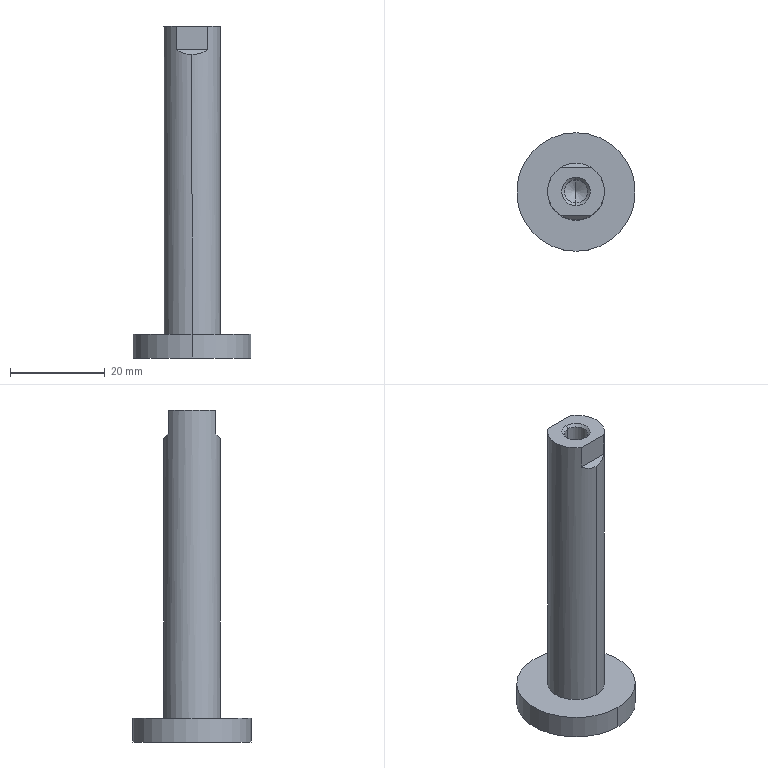Component | SolidWorks | CDQ2B25-50DZ-M9N(0_0_0)-1_CDQ2B25-50M9N(0_0)_CYROD-1 | 1 solid | 17 faces | box 25 x 25 x 70 mm | volume 9518 mm3 | plane 7 | cylinder 6 | cone 4 | commonest cylinder face diameters 25 x2 12 x2 4.917 x2
build123d program:
from build123d import *

# Parameters (mm, degrees)
EXTRUDE1_DEPTH      = 12
EXTRUDE1_DEPTH_BACK = 12


with BuildPart() as part:
    # Sketch1 → Revolve1 (revolve)
    with BuildSketch(Plane.XY, mode=Mode.PRIVATE) as revolve1_sk:
        Polygon((8.419, 0), (7, 2.458), (-4.458, 2.458), (-5, 3), (-5, 6), (60, 6), (60, 12.5), (65, 12.5), (65, 0), align=None)
    revolve(revolve1_sk.sketch.rotate(Axis((65, 0, 0), (-1, 0, 0)), 270), axis=Axis((65, 0, 0), (-1, 0, 0)))

    # Sketch2 → Extrude1 (cut, two sides: drawn at the far end of the back side and taken through both)
    with BuildSketch(Plane(origin=(0, 0, 0), x_dir=(1, 0, 0), z_dir=(0, 1, 0)).offset(-EXTRUDE1_DEPTH_BACK)):
        Polygon((-10, 10), (-10, -10), (5, -10), (0, -5), (-5, -5), (-5, 5), (0, 5), (5, 10), align=None)
    extrude(amount=EXTRUDE1_DEPTH + EXTRUDE1_DEPTH_BACK, mode=Mode.SUBTRACT)


solid = part.part

# Placed as in the assembly
solid = solid.moved(Location((0, -65.5, 248.966), (90, 0, -90)))
STEP:
#1=COLOUR_RGB('',0.7922,0.8196,0.9333);
#2=FILL_AREA_STYLE_COLOUR('',#1);
#3=FILL_AREA_STYLE('',(#2));
#4=SURFACE_STYLE_FILL_AREA(#3);
#5=SURFACE_SIDE_STYLE('',(#4));
#6=SURFACE_STYLE_USAGE(.BOTH.,#5);
#7=PRESENTATION_STYLE_ASSIGNMENT((#6));
#8=CARTESIAN_POINT('',(-0.,-3.071,7.243));
#9=VERTEX_POINT('',#8);
#10=CARTESIAN_POINT('',(-0.,-2.087,7.243));
#11=VERTEX_POINT('',#10);
#12=CARTESIAN_POINT('',(-0.,-2.579,7.243));
#13=DIRECTION('',(-0.,0.,1.));
#14=DIRECTION('',(0.,-1.,0.));
#15=AXIS2_PLACEMENT_3D('',#12,#13,#14);
#16=CIRCLE('',#15,0.4921);
#17=EDGE_CURVE('',#9,#11,#16,.T.);
#18=ORIENTED_EDGE('',*,*,#17,.T.);
#19=CARTESIAN_POINT('',(-0.,-2.087,7.44));
#20=VERTEX_POINT('',#19);
#21=CARTESIAN_POINT('',(-0.,-2.087,7.243));
#22=DIRECTION('',(-0.,0.,1.));
#23=VECTOR('',#22,39.37);
#24=LINE('',#21,#23);
#25=EDGE_CURVE('',#11,#20,#24,.T.);
#26=ORIENTED_EDGE('',*,*,#25,.T.);
#27=CARTESIAN_POINT('',(-0.,-3.071,7.44));
#28=VERTEX_POINT('',#27);
#29=CARTESIAN_POINT('',(-0.,-2.579,7.44));
#30=DIRECTION('',(-0.,0.,1.));
#31=DIRECTION('',(0.,-1.,0.));
#32=AXIS2_PLACEMENT_3D('',#29,#30,#31);
#33=CIRCLE('',#32,0.4921);
#34=EDGE_CURVE('',#28,#20,#33,.T.);
#35=ORIENTED_EDGE('',*,*,#34,.F.);
#36=CARTESIAN_POINT('',(-0.,-3.071,7.243));
#37=DIRECTION('',(-0.,0.,1.));
#38=VECTOR('',#37,39.37);
#39=LINE('',#36,#38);
#40=EDGE_CURVE('',#9,#28,#39,.T.);
#41=ORIENTED_EDGE('',*,*,#40,.F.);
#42=EDGE_LOOP('',(#18,#26,#35,#41));
#43=FACE_OUTER_BOUND('',#42,.T.);
#44=CARTESIAN_POINT('',(-0.,-2.579,7.243));
#45=DIRECTION('',(-0.,0.,1.));
#46=DIRECTION('',(0.,-1.,0.));
#47=AXIS2_PLACEMENT_3D('',#44,#45,#46);
#48=CYLINDRICAL_SURFACE('',#47,0.4921);
#49=ADVANCED_FACE('',(#43),#48,.T.);
#50=CARTESIAN_POINT('',(-0.,-2.815,7.44));
#51=VERTEX_POINT('',#50);
#52=CARTESIAN_POINT('',(-0.,-2.343,7.44));
#53=VERTEX_POINT('',#52);
#54=CARTESIAN_POINT('',(-0.,-2.579,7.44));
#55=DIRECTION('',(-0.,0.,1.));
#56=DIRECTION('',(0.,-1.,0.));
#57=AXIS2_PLACEMENT_3D('',#54,#55,#56);
#58=CIRCLE('',#57,0.2362);
#59=EDGE_CURVE('',#51,#53,#58,.T.);
#60=ORIENTED_EDGE('',*,*,#59,.T.);
#61=CARTESIAN_POINT('',(-0.,-2.343,9.762));
#62=VERTEX_POINT('',#61);
#63=CARTESIAN_POINT('',(-0.,-2.343,7.243));
#64=DIRECTION('',(-0.,0.,1.));
#65=VECTOR('',#64,39.37);
#66=LINE('',#63,#65);
#67=EDGE_CURVE('',#53,#62,#66,.T.);
#68=ORIENTED_EDGE('',*,*,#67,.T.);
#69=CARTESIAN_POINT('',(0.1306,-2.382,9.802));
#70=VERTEX_POINT('',#69);
#71=CARTESIAN_POINT('',(-0.,-2.343,9.762));
#72=CARTESIAN_POINT('',(0.04679,-2.343,9.762));
#73=CARTESIAN_POINT('',(0.09159,-2.356,9.776));
#74=CARTESIAN_POINT('',(0.1306,-2.382,9.802));
#75=(BOUNDED_CURVE()B_SPLINE_CURVE(3,(#71,#72,#73,#74),.UNSPECIFIED.,.F.,.T.)B_SPLINE_CURVE_WITH_KNOTS((4,4),(3.142,3.727),.UNSPECIFIED.)CURVE()GEOMETRIC_REPRESENTATION_ITEM()RATIONAL_B_SPLINE_CURVE((1.,0.9716,0.9716,1.))REPRESENTATION_ITEM(''));
#76=EDGE_CURVE('',#62,#70,#75,.T.);
#77=ORIENTED_EDGE('',*,*,#76,.T.);
#78=CARTESIAN_POINT('',(0.1306,-2.382,9.999));
#79=VERTEX_POINT('',#78);
#80=CARTESIAN_POINT('',(0.1306,-2.382,7.243));
#81=DIRECTION('',(-0.,0.,1.));
#82=VECTOR('',#81,39.37);
#83=LINE('',#80,#82);
#84=EDGE_CURVE('',#70,#79,#83,.T.);
#85=ORIENTED_EDGE('',*,*,#84,.T.);
#86=CARTESIAN_POINT('',(0.1306,-2.776,9.999));
#87=VERTEX_POINT('',#86);
#88=CARTESIAN_POINT('',(-0.,-2.579,9.999));
#89=DIRECTION('',(-0.,0.,1.));
#90=DIRECTION('',(0.,-1.,0.));
#91=AXIS2_PLACEMENT_3D('',#88,#89,#90);
#92=CIRCLE('',#91,0.2362);
#93=EDGE_CURVE('',#87,#79,#92,.T.);
#94=ORIENTED_EDGE('',*,*,#93,.F.);
#95=CARTESIAN_POINT('',(0.1306,-2.776,9.802));
#96=VERTEX_POINT('',#95);
#97=CARTESIAN_POINT('',(0.1306,-2.776,7.243));
#98=DIRECTION('',(0.,-0.,-1.));
#99=VECTOR('',#98,39.37);
#100=LINE('',#97,#99);
#101=EDGE_CURVE('',#87,#96,#100,.T.);
#102=ORIENTED_EDGE('',*,*,#101,.T.);
#103=CARTESIAN_POINT('',(-0.,-2.815,9.762));
#104=VERTEX_POINT('',#103);
#105=CARTESIAN_POINT('',(0.1306,-2.776,9.802));
#106=CARTESIAN_POINT('',(0.09159,-2.801,9.776));
#107=CARTESIAN_POINT('',(0.04679,-2.815,9.762));
#108=CARTESIAN_POINT('',(-0.,-2.815,9.762));
#109=(BOUNDED_CURVE()B_SPLINE_CURVE(3,(#105,#106,#107,#108),.UNSPECIFIED.,.F.,.T.)B_SPLINE_CURVE_WITH_KNOTS((4,4),(2.556,3.142),.UNSPECIFIED.)CURVE()GEOMETRIC_REPRESENTATION_ITEM()RATIONAL_B_SPLINE_CURVE((1.,0.9716,0.9716,1.))REPRESENTATION_ITEM(''));
#110=EDGE_CURVE('',#96,#104,#109,.T.);
#111=ORIENTED_EDGE('',*,*,#110,.T.);
#112=CARTESIAN_POINT('',(-0.,-2.815,7.243));
#113=DIRECTION('',(-0.,0.,1.));
#114=VECTOR('',#113,39.37);
#115=LINE('',#112,#114);
#116=EDGE_CURVE('',#51,#104,#115,.T.);
#117=ORIENTED_EDGE('',*,*,#116,.F.);
#118=EDGE_LOOP('',(#60,#68,#77,#85,#94,#102,#111,#117));
#119=FACE_OUTER_BOUND('',#118,.T.);
#120=CARTESIAN_POINT('',(-0.,-2.579,7.243));
#121=DIRECTION('',(-0.,0.,1.));
#122=DIRECTION('',(0.,-1.,0.));
#123=AXIS2_PLACEMENT_3D('',#120,#121,#122);
#124=CYLINDRICAL_SURFACE('',#123,0.2362);
#125=ADVANCED_FACE('',(#119),#124,.T.);
#126=CARTESIAN_POINT('',(-0.,-2.482,9.977));
#127=VERTEX_POINT('',#126);
#128=CARTESIAN_POINT('',(-0.,-2.676,9.977));
#129=VERTEX_POINT('',#128);
#130=CARTESIAN_POINT('',(-0.,-2.579,9.977));
#131=DIRECTION('',(-0.,0.,1.));
#132=DIRECTION('',(0.,-1.,0.));
#133=AXIS2_PLACEMENT_3D('',#130,#131,#132);
#134=CIRCLE('',#133,0.09679);
#135=EDGE_CURVE('',#127,#129,#134,.T.);
#136=ORIENTED_EDGE('',*,*,#135,.F.);
#137=CARTESIAN_POINT('',(-0.,-2.461,9.999));
#138=VERTEX_POINT('',#137);
#139=CARTESIAN_POINT('',(-0.,-2.461,9.999));
#140=DIRECTION('',(-0.,0.7071,0.7071));
#141=VECTOR('',#140,39.37);
#142=LINE('',#139,#141);
#143=EDGE_CURVE('',#127,#138,#142,.T.);
#144=ORIENTED_EDGE('',*,*,#143,.T.);
#145=CARTESIAN_POINT('',(-0.,-2.697,9.999));
#146=VERTEX_POINT('',#145);
#147=CARTESIAN_POINT('',(-0.,-2.579,9.999));
#148=DIRECTION('',(-0.,0.,1.));
#149=DIRECTION('',(0.,-1.,0.));
#150=AXIS2_PLACEMENT_3D('',#147,#148,#149);
#151=CIRCLE('',#150,0.1181);
#152=EDGE_CURVE('',#138,#146,#151,.T.);
#153=ORIENTED_EDGE('',*,*,#152,.T.);
#154=CARTESIAN_POINT('',(-0.,-2.697,9.999));
#155=DIRECTION('',(0.,-0.7071,0.7071));
#156=VECTOR('',#155,39.37);
#157=LINE('',#154,#156);
#158=EDGE_CURVE('',#129,#146,#157,.T.);
#159=ORIENTED_EDGE('',*,*,#158,.F.);
#160=EDGE_LOOP('',(#136,#144,#153,#159));
#161=FACE_OUTER_BOUND('',#160,.T.);
#162=CARTESIAN_POINT('',(-0.,-2.579,9.999));
#163=DIRECTION('',(-0.,0.,1.));
#164=DIRECTION('',(0.,-1.,0.));
#165=AXIS2_PLACEMENT_3D('',#162,#163,#164);
#166=CONICAL_SURFACE('',#165,0.1181,0.7854);
#167=ADVANCED_FACE('',(#161),#166,.F.);
#168=CARTESIAN_POINT('',(-0.,-2.482,9.526));
#169=VERTEX_POINT('',#168);
#170=CARTESIAN_POINT('',(-0.,-2.676,9.526));
#171=VERTEX_POINT('',#170);
#172=CARTESIAN_POINT('',(-0.,-2.579,9.526));
#173=DIRECTION('',(-0.,0.,1.));
#174=DIRECTION('',(0.,-1.,0.));
#175=AXIS2_PLACEMENT_3D('',#172,#173,#174);
#176=CIRCLE('',#175,0.09679);
#177=EDGE_CURVE('',#169,#171,#176,.T.);
#178=ORIENTED_EDGE('',*,*,#177,.F.);
#179=CARTESIAN_POINT('',(-0.,-2.482,7.243));
#180=DIRECTION('',(-0.,0.,1.));
#181=VECTOR('',#180,39.37);
#182=LINE('',#179,#181);
#183=EDGE_CURVE('',#169,#127,#182,.T.);
#184=ORIENTED_EDGE('',*,*,#183,.T.);
#185=ORIENTED_EDGE('',*,*,#135,.T.);
#186=CARTESIAN_POINT('',(-0.,-2.676,7.243));
#187=DIRECTION('',(-0.,0.,1.));
#188=VECTOR('',#187,39.37);
#189=LINE('',#186,#188);
#190=EDGE_CURVE('',#171,#129,#189,.T.);
#191=ORIENTED_EDGE('',*,*,#190,.F.);
#192=EDGE_LOOP('',(#178,#184,#185,#191));
#193=FACE_OUTER_BOUND('',#192,.T.);
#194=CARTESIAN_POINT('',(-0.,-2.579,7.243));
#195=DIRECTION('',(-0.,0.,1.));
#196=DIRECTION('',(0.,-1.,0.));
#197=AXIS2_PLACEMENT_3D('',#194,#195,#196);
#198=CYLINDRICAL_SURFACE('',#197,0.09679);
#199=ADVANCED_FACE('',(#193),#198,.F.);
#200=CARTESIAN_POINT('',(-0.,-2.579,9.47));
#201=VERTEX_POINT('',#200);
#202=CARTESIAN_POINT('',(-0.,-2.676,9.526));
#203=DIRECTION('',(0.,-0.866,0.5));
#204=VECTOR('',#203,39.37);
#205=LINE('',#202,#204);
#206=EDGE_CURVE('',#201,#171,#205,.T.);
#207=ORIENTED_EDGE('',*,*,#206,.F.);
#208=CARTESIAN_POINT('',(-0.,-2.482,9.526));
#209=DIRECTION('',(-0.,0.866,0.5));
#210=VECTOR('',#209,39.37);
#211=LINE('',#208,#210);
#212=EDGE_CURVE('',#201,#169,#211,.T.);
#213=ORIENTED_EDGE('',*,*,#212,.T.);
#214=ORIENTED_EDGE('',*,*,#177,.T.);
#215=EDGE_LOOP('',(#207,#213,#214));
#216=FACE_OUTER_BOUND('',#215,.T.);
#217=CARTESIAN_POINT('',(-0.,-2.579,9.526));
#218=DIRECTION('',(-0.,0.,1.));
#219=DIRECTION('',(0.,-1.,0.));
#220=AXIS2_PLACEMENT_3D('',#217,#218,#219);
#221=CONICAL_SURFACE('',#220,0.09679,1.047);
#222=ADVANCED_FACE('',(#216),#221,.F.);
#223=ORIENTED_EDGE('',*,*,#212,.F.);
#224=ORIENTED_EDGE('',*,*,#206,.T.);
#225=CARTESIAN_POINT('',(-0.,-2.579,9.526));
#226=DIRECTION('',(-0.,0.,1.));
#227=DIRECTION('',(0.,-1.,0.));
#228=AXIS2_PLACEMENT_3D('',#225,#226,#227);
#229=CIRCLE('',#228,0.09679);
#230=EDGE_CURVE('',#171,#169,#229,.T.);
#231=ORIENTED_EDGE('',*,*,#230,.T.);
#232=EDGE_LOOP('',(#223,#224,#231));
#233=FACE_OUTER_BOUND('',#232,.T.);
#234=CARTESIAN_POINT('',(-0.,-2.579,9.526));
#235=DIRECTION('',(-0.,0.,1.));
#236=DIRECTION('',(0.,-1.,0.));
#237=AXIS2_PLACEMENT_3D('',#234,#235,#236);
#238=CONICAL_SURFACE('',#237,0.09679,1.047);
#239=ADVANCED_FACE('',(#233),#238,.F.);
#240=ORIENTED_EDGE('',*,*,#183,.F.);
#241=ORIENTED_EDGE('',*,*,#230,.F.);
#242=ORIENTED_EDGE('',*,*,#190,.T.);
#243=CARTESIAN_POINT('',(-0.,-2.579,9.977));
#244=DIRECTION('',(-0.,0.,1.));
#245=DIRECTION('',(0.,-1.,0.));
#246=AXIS2_PLACEMENT_3D('',#243,#244,#245);
#247=CIRCLE('',#246,0.09679);
#248=EDGE_CURVE('',#129,#127,#247,.T.);
#249=ORIENTED_EDGE('',*,*,#248,.T.);
#250=EDGE_LOOP('',(#240,#241,#242,#249));
#251=FACE_OUTER_BOUND('',#250,.T.);
#252=CARTESIAN_POINT('',(-0.,-2.579,7.243));
#253=DIRECTION('',(-0.,0.,1.));
#254=DIRECTION('',(0.,-1.,0.));
#255=AXIS2_PLACEMENT_3D('',#252,#253,#254);
#256=CYLINDRICAL_SURFACE('',#255,0.09679);
#257=ADVANCED_FACE('',(#251),#256,.F.);
#258=ORIENTED_EDGE('',*,*,#143,.F.);
#259=ORIENTED_EDGE('',*,*,#248,.F.);
#260=ORIENTED_EDGE('',*,*,#158,.T.);
#261=CARTESIAN_POINT('',(-0.,-2.579,9.999));
#262=DIRECTION('',(-0.,0.,1.));
#263=DIRECTION('',(0.,-1.,0.));
#264=AXIS2_PLACEMENT_3D('',#261,#262,#263);
#265=CIRCLE('',#264,0.1181);
#266=EDGE_CURVE('',#146,#138,#265,.T.);
#267=ORIENTED_EDGE('',*,*,#266,.T.);
#268=EDGE_LOOP('',(#258,#259,#260,#267));
#269=FACE_OUTER_BOUND('',#268,.T.);
#270=CARTESIAN_POINT('',(-0.,-2.579,9.999));
#271=DIRECTION('',(-0.,0.,1.));
#272=DIRECTION('',(0.,-1.,0.));
#273=AXIS2_PLACEMENT_3D('',#270,#271,#272);
#274=CONICAL_SURFACE('',#273,0.1181,0.7854);
#275=ADVANCED_FACE('',(#269),#274,.F.);
#276=ORIENTED_EDGE('',*,*,#266,.F.);
#277=ORIENTED_EDGE('',*,*,#152,.F.);
#278=EDGE_LOOP('',(#276,#277));
#279=FACE_BOUND('',#278,.T.);
#280=ORIENTED_EDGE('',*,*,#93,.T.);
#281=CARTESIAN_POINT('',(-0.1306,-2.382,9.999));
#282=VERTEX_POINT('',#281);
#283=CARTESIAN_POINT('',(-0.4724,-2.382,9.999));
#284=DIRECTION('',(1.,0.,0.));
#285=VECTOR('',#284,39.37);
#286=LINE('',#283,#285);
#287=EDGE_CURVE('',#282,#79,#286,.T.);
#288=ORIENTED_EDGE('',*,*,#287,.F.);
#289=CARTESIAN_POINT('',(-0.1306,-2.776,9.999));
#290=VERTEX_POINT('',#289);
#291=CARTESIAN_POINT('',(-0.,-2.579,9.999));
#292=DIRECTION('',(-0.,0.,1.));
#293=DIRECTION('',(0.,-1.,0.));
#294=AXIS2_PLACEMENT_3D('',#291,#292,#293);
#295=CIRCLE('',#294,0.2362);
#296=EDGE_CURVE('',#282,#290,#295,.T.);
#297=ORIENTED_EDGE('',*,*,#296,.T.);
#298=CARTESIAN_POINT('',(-0.4724,-2.776,9.999));
#299=DIRECTION('',(1.,0.,0.));
#300=VECTOR('',#299,39.37);
#301=LINE('',#298,#300);
#302=EDGE_CURVE('',#290,#87,#301,.T.);
#303=ORIENTED_EDGE('',*,*,#302,.T.);
#304=EDGE_LOOP('',(#280,#288,#297,#303));
#305=FACE_OUTER_BOUND('',#304,.T.);
#306=CARTESIAN_POINT('',(0.1181,-2.579,9.999));
#307=DIRECTION('',(0.,-0.,-1.));
#308=DIRECTION('',(-0.,1.,-0.));
#309=AXIS2_PLACEMENT_3D('',#306,#307,#308);
#310=PLANE('',#309);
#311=ADVANCED_FACE('',(#279,#305),#310,.F.);
#312=ORIENTED_EDGE('',*,*,#67,.F.);
#313=CARTESIAN_POINT('',(-0.,-2.579,7.44));
#314=DIRECTION('',(-0.,0.,1.));
#315=DIRECTION('',(0.,-1.,0.));
#316=AXIS2_PLACEMENT_3D('',#313,#314,#315);
#317=CIRCLE('',#316,0.2362);
#318=EDGE_CURVE('',#53,#51,#317,.T.);
#319=ORIENTED_EDGE('',*,*,#318,.T.);
#320=ORIENTED_EDGE('',*,*,#116,.T.);
#321=CARTESIAN_POINT('',(-0.1306,-2.776,9.802));
#322=VERTEX_POINT('',#321);
#323=CARTESIAN_POINT('',(-0.,-2.815,9.762));
#324=CARTESIAN_POINT('',(-0.04679,-2.815,9.762));
#325=CARTESIAN_POINT('',(-0.09159,-2.801,9.776));
#326=CARTESIAN_POINT('',(-0.1306,-2.776,9.802));
#327=(BOUNDED_CURVE()B_SPLINE_CURVE(3,(#323,#324,#325,#326),.UNSPECIFIED.,.F.,.T.)B_SPLINE_CURVE_WITH_KNOTS((4,4),(3.142,3.727),.UNSPECIFIED.)CURVE()GEOMETRIC_REPRESENTATION_ITEM()RATIONAL_B_SPLINE_CURVE((1.,0.9716,0.9716,1.))REPRESENTATION_ITEM(''));
#328=EDGE_CURVE('',#104,#322,#327,.T.);
#329=ORIENTED_EDGE('',*,*,#328,.T.);
#330=CARTESIAN_POINT('',(-0.1306,-2.776,7.243));
#331=DIRECTION('',(-0.,0.,1.));
#332=VECTOR('',#331,39.37);
#333=LINE('',#330,#332);
#334=EDGE_CURVE('',#322,#290,#333,.T.);
#335=ORIENTED_EDGE('',*,*,#334,.T.);
#336=ORIENTED_EDGE('',*,*,#296,.F.);
#337=CARTESIAN_POINT('',(-0.1306,-2.382,9.802));
#338=VERTEX_POINT('',#337);
#339=CARTESIAN_POINT('',(-0.1306,-2.382,7.243));
#340=DIRECTION('',(0.,-0.,-1.));
#341=VECTOR('',#340,39.37);
#342=LINE('',#339,#341);
#343=EDGE_CURVE('',#282,#338,#342,.T.);
#344=ORIENTED_EDGE('',*,*,#343,.T.);
#345=CARTESIAN_POINT('',(-0.1306,-2.382,9.802));
#346=CARTESIAN_POINT('',(-0.09159,-2.356,9.776));
#347=CARTESIAN_POINT('',(-0.04679,-2.343,9.762));
#348=CARTESIAN_POINT('',(-0.,-2.343,9.762));
#349=(BOUNDED_CURVE()B_SPLINE_CURVE(3,(#345,#346,#347,#348),.UNSPECIFIED.,.F.,.T.)B_SPLINE_CURVE_WITH_KNOTS((4,4),(2.556,3.142),.UNSPECIFIED.)CURVE()GEOMETRIC_REPRESENTATION_ITEM()RATIONAL_B_SPLINE_CURVE((1.,0.9716,0.9716,1.))REPRESENTATION_ITEM(''));
#350=EDGE_CURVE('',#338,#62,#349,.T.);
#351=ORIENTED_EDGE('',*,*,#350,.T.);
#352=EDGE_LOOP('',(#312,#319,#320,#329,#335,#336,#344,#351));
#353=FACE_OUTER_BOUND('',#352,.T.);
#354=CARTESIAN_POINT('',(-0.,-2.579,7.243));
#355=DIRECTION('',(-0.,0.,1.));
#356=DIRECTION('',(0.,-1.,0.));
#357=AXIS2_PLACEMENT_3D('',#354,#355,#356);
#358=CYLINDRICAL_SURFACE('',#357,0.2362);
#359=ADVANCED_FACE('',(#353),#358,.T.);
#360=ORIENTED_EDGE('',*,*,#59,.F.);
#361=ORIENTED_EDGE('',*,*,#318,.F.);
#362=EDGE_LOOP('',(#360,#361));
#363=FACE_BOUND('',#362,.T.);
#364=ORIENTED_EDGE('',*,*,#34,.T.);
#365=CARTESIAN_POINT('',(-0.,-2.579,7.44));
#366=DIRECTION('',(-0.,0.,1.));
#367=DIRECTION('',(0.,-1.,0.));
#368=AXIS2_PLACEMENT_3D('',#365,#366,#367);
#369=CIRCLE('',#368,0.4921);
#370=EDGE_CURVE('',#20,#28,#369,.T.);
#371=ORIENTED_EDGE('',*,*,#370,.T.);
#372=EDGE_LOOP('',(#364,#371));
#373=FACE_OUTER_BOUND('',#372,.T.);
#374=CARTESIAN_POINT('',(0.2362,-2.579,7.44));
#375=DIRECTION('',(0.,-0.,-1.));
#376=DIRECTION('',(-0.,1.,-0.));
#377=AXIS2_PLACEMENT_3D('',#374,#375,#376);
#378=PLANE('',#377);
#379=ADVANCED_FACE('',(#363,#373),#378,.F.);
#380=ORIENTED_EDGE('',*,*,#25,.F.);
#381=CARTESIAN_POINT('',(-0.,-2.579,7.243));
#382=DIRECTION('',(-0.,0.,1.));
#383=DIRECTION('',(0.,-1.,0.));
#384=AXIS2_PLACEMENT_3D('',#381,#382,#383);
#385=CIRCLE('',#384,0.4921);
#386=EDGE_CURVE('',#11,#9,#385,.T.);
#387=ORIENTED_EDGE('',*,*,#386,.T.);
#388=ORIENTED_EDGE('',*,*,#40,.T.);
#389=ORIENTED_EDGE('',*,*,#370,.F.);
#390=EDGE_LOOP('',(#380,#387,#388,#389));
#391=FACE_OUTER_BOUND('',#390,.T.);
#392=CARTESIAN_POINT('',(-0.,-2.579,7.243));
#393=DIRECTION('',(-0.,0.,1.));
#394=DIRECTION('',(0.,-1.,0.));
#395=AXIS2_PLACEMENT_3D('',#392,#393,#394);
#396=CYLINDRICAL_SURFACE('',#395,0.4921);
#397=ADVANCED_FACE('',(#391),#396,.T.);
#398=ORIENTED_EDGE('',*,*,#17,.F.);
#399=ORIENTED_EDGE('',*,*,#386,.F.);
#400=EDGE_LOOP('',(#398,#399));
#401=FACE_OUTER_BOUND('',#400,.T.);
#402=CARTESIAN_POINT('',(0.4921,-2.579,7.243));
#403=DIRECTION('',(-0.,0.,1.));
#404=DIRECTION('',(0.,-1.,0.));
#405=AXIS2_PLACEMENT_3D('',#402,#403,#404);
#406=PLANE('',#405);
#407=ADVANCED_FACE('',(#401),#406,.F.);
#408=CARTESIAN_POINT('',(-0.4724,-2.776,9.802));
#409=DIRECTION('',(1.,0.,0.));
#410=VECTOR('',#409,39.37);
#411=LINE('',#408,#410);
#412=EDGE_CURVE('',#322,#96,#411,.T.);
#413=ORIENTED_EDGE('',*,*,#412,.F.);
#414=ORIENTED_EDGE('',*,*,#328,.F.);
#415=ORIENTED_EDGE('',*,*,#110,.F.);
#416=EDGE_LOOP('',(#413,#414,#415));
#417=FACE_OUTER_BOUND('',#416,.T.);
#418=CARTESIAN_POINT('',(-0.4724,-2.972,9.605));
#419=DIRECTION('',(-0.,0.7071,-0.7071));
#420=DIRECTION('',(-0.,0.7071,0.7071));
#421=AXIS2_PLACEMENT_3D('',#418,#419,#420);
#422=PLANE('',#421);
#423=ADVANCED_FACE('',(#417),#422,.F.);
#424=ORIENTED_EDGE('',*,*,#412,.T.);
#425=ORIENTED_EDGE('',*,*,#101,.F.);
#426=ORIENTED_EDGE('',*,*,#302,.F.);
#427=ORIENTED_EDGE('',*,*,#334,.F.);
#428=EDGE_LOOP('',(#424,#425,#426,#427));
#429=FACE_OUTER_BOUND('',#428,.T.);
#430=CARTESIAN_POINT('',(-0.4724,-2.776,9.802));
#431=DIRECTION('',(-0.,1.,-0.));
#432=DIRECTION('',(-0.,0.,1.));
#433=AXIS2_PLACEMENT_3D('',#430,#431,#432);
#434=PLANE('',#433);
#435=ADVANCED_FACE('',(#429),#434,.F.);
#436=CARTESIAN_POINT('',(-0.4724,-2.382,9.802));
#437=DIRECTION('',(1.,0.,0.));
#438=VECTOR('',#437,39.37);
#439=LINE('',#436,#438);
#440=EDGE_CURVE('',#338,#70,#439,.T.);
#441=ORIENTED_EDGE('',*,*,#440,.T.);
#442=ORIENTED_EDGE('',*,*,#76,.F.);
#443=ORIENTED_EDGE('',*,*,#350,.F.);
#444=EDGE_LOOP('',(#441,#442,#443));
#445=FACE_OUTER_BOUND('',#444,.T.);
#446=CARTESIAN_POINT('',(-0.4724,-2.382,9.802));
#447=DIRECTION('',(0.,-0.7071,-0.7071));
#448=DIRECTION('',(-0.,0.7071,-0.7071));
#449=AXIS2_PLACEMENT_3D('',#446,#447,#448);
#450=PLANE('',#449);
#451=ADVANCED_FACE('',(#445),#450,.F.);
#452=ORIENTED_EDGE('',*,*,#440,.F.);
#453=ORIENTED_EDGE('',*,*,#343,.F.);
#454=ORIENTED_EDGE('',*,*,#287,.T.);
#455=ORIENTED_EDGE('',*,*,#84,.F.);
#456=EDGE_LOOP('',(#452,#453,#454,#455));
#457=FACE_OUTER_BOUND('',#456,.T.);
#458=CARTESIAN_POINT('',(-0.4724,-2.382,9.999));
#459=DIRECTION('',(0.,-1.,0.));
#460=DIRECTION('',(0.,-0.,-1.));
#461=AXIS2_PLACEMENT_3D('',#458,#459,#460);
#462=PLANE('',#461);
#463=ADVANCED_FACE('',(#457),#462,.F.);
#464=CLOSED_SHELL('',(#49,#125,#167,#199,#222,#239,#257,#275,#311,#359,#379,#397,#407,#423,#435,#451,#463));
#465=MANIFOLD_SOLID_BREP('',#464);
#466=STYLED_ITEM('',(#7),#465);
#467=PRESENTATION_LAYER_ASSIGNMENT('','',(#466));
#468=(LENGTH_UNIT()NAMED_UNIT(*)SI_UNIT($,.METRE.));
#469=LENGTH_MEASURE_WITH_UNIT(LENGTH_MEASURE(0.0254),#468);
#470=DIMENSIONAL_EXPONENTS(1.,0.,0.,0.,0.,0.,0.);
#471=(CONVERSION_BASED_UNIT('',#469)LENGTH_UNIT()NAMED_UNIT(#470));
#472=UNCERTAINTY_MEASURE_WITH_UNIT(LENGTH_MEASURE(0.00001),#471,'','');
#473=(NAMED_UNIT(*)PLANE_ANGLE_UNIT()SI_UNIT($,.RADIAN.));
#474=(NAMED_UNIT(*)SI_UNIT($,.STERADIAN.)SOLID_ANGLE_UNIT());
#475=(GEOMETRIC_REPRESENTATION_CONTEXT(3)GLOBAL_UNCERTAINTY_ASSIGNED_CONTEXT((#472))GLOBAL_UNIT_ASSIGNED_CONTEXT((#471,#473,#474))REPRESENTATION_CONTEXT('',''));
#476=MECHANICAL_DESIGN_GEOMETRIC_PRESENTATION_REPRESENTATION('',(#466),#475);
#477=CARTESIAN_POINT('',(0.,0.,0.));
#478=DIRECTION('',(0.,0.,1.));
#479=DIRECTION('',(1.,0.,0.));
#480=AXIS2_PLACEMENT_3D('',#477,#478,#479);
#481=(LENGTH_UNIT()NAMED_UNIT(*)SI_UNIT($,.METRE.));
#482=LENGTH_MEASURE_WITH_UNIT(LENGTH_MEASURE(0.0254),#481);
#483=DIMENSIONAL_EXPONENTS(1.,0.,0.,0.,0.,0.,0.);
#484=(CONVERSION_BASED_UNIT('',#482)LENGTH_UNIT()NAMED_UNIT(#483));
#485=UNCERTAINTY_MEASURE_WITH_UNIT(LENGTH_MEASURE(0.00001),#484,'','');
#486=(NAMED_UNIT(*)PLANE_ANGLE_UNIT()SI_UNIT($,.RADIAN.));
#487=(NAMED_UNIT(*)SI_UNIT($,.STERADIAN.)SOLID_ANGLE_UNIT());
#488=(GEOMETRIC_REPRESENTATION_CONTEXT(3)GLOBAL_UNCERTAINTY_ASSIGNED_CONTEXT((#485))GLOBAL_UNIT_ASSIGNED_CONTEXT((#484,#486,#487))REPRESENTATION_CONTEXT('',''));
#489=ADVANCED_BREP_SHAPE_REPRESENTATION('',(#465,#480),#488);